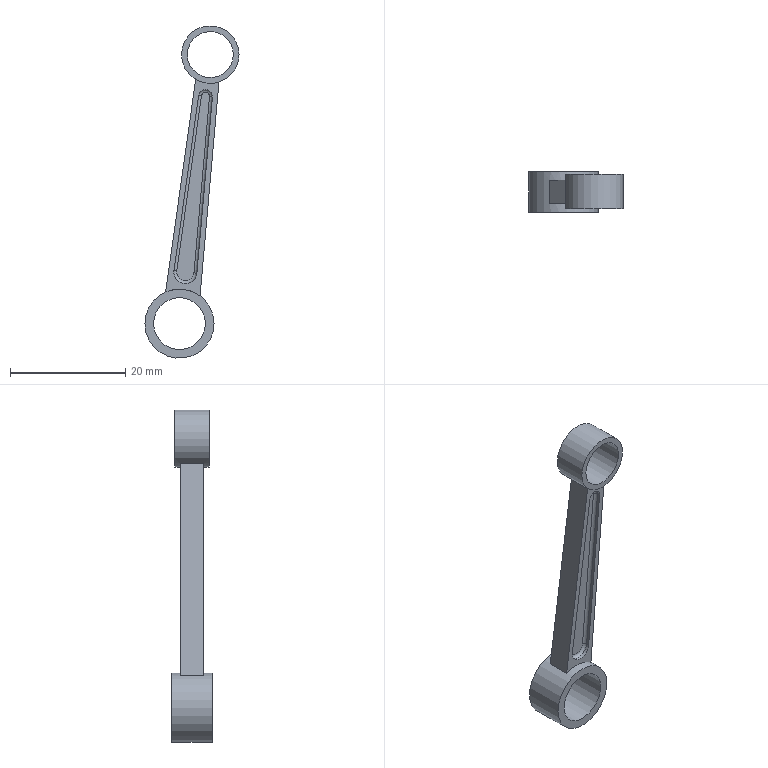Component | NX | CON_ROD | 1 solid | 30 faces | volume 1041 mm3 | plane 14 | cylinder 12 | torus 4 | commonest cylinder face diameters 1 x4 4 x2 2.4 x2 10 x1 12 x1 8 x1 9 x1